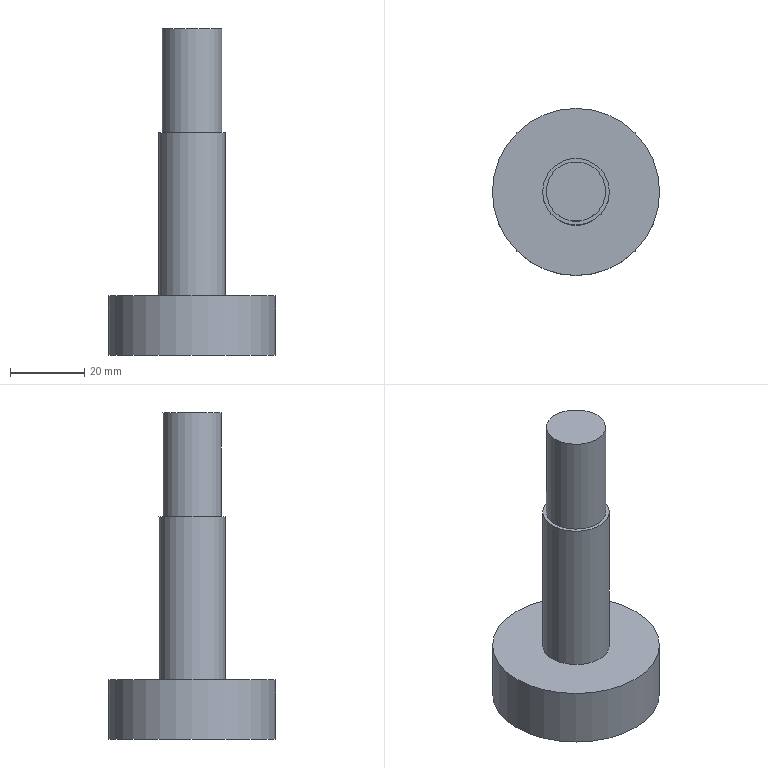Component | NX | VALVE_CORE | 1 solid | 7 faces | box 45 x 45 x 88 mm | volume 42273 mm3 | plane 4 | cylinder 3 | commonest cylinder face diameters 45 x1 18 x1 16 x1
STEP:
#1=CARTESIAN_POINT('',(0.,0.,0.));
#2=DIRECTION('',(0.,0.,1.));
#3=DIRECTION('',(1.,0.,0.));
#4=AXIS2_PLACEMENT_3D('',#1,#2,#3);
#5=CARTESIAN_POINT('',(90.249,-116.649,-76.615));
#6=VERTEX_POINT('',#5);
#7=CARTESIAN_POINT('',(81.249,-116.649,-76.615));
#8=DIRECTION('',(0.,0.,1.));
#9=DIRECTION('',(1.,0.,0.));
#10=AXIS2_PLACEMENT_3D('',#7,#8,#9);
#11=CIRCLE('',#10,9.);
#12=CARTESIAN_POINT('',(81.249,-116.649,-76.615));
#13=DIRECTION('',(0.,0.,1.));
#14=DIRECTION('',(1.,0.,0.));
#15=AXIS2_PLACEMENT_3D('',#12,#13,#14);
#16=PLANE('',#15);
#17=CARTESIAN_POINT('',(0.,0.));
#18=DIRECTION('',(1.,0.));
#19=AXIS2_PLACEMENT_2D('',#17,#18);
#20=CIRCLE('',#19,9.);
#21=(GEOMETRIC_REPRESENTATION_CONTEXT(2)PARAMETRIC_REPRESENTATION_CONTEXT()REPRESENTATION_CONTEXT('',''));
#22=DEFINITIONAL_REPRESENTATION('',(#20),#21);
#23=PCURVE('',#16,#22);
#24=CARTESIAN_POINT('',(81.249,-116.649,-76.615));
#25=DIRECTION('',(0.,0.,1.));
#26=DIRECTION('',(1.,0.,0.));
#27=AXIS2_PLACEMENT_3D('',#24,#25,#26);
#28=CYLINDRICAL_SURFACE('',#27,9.);
#29=CARTESIAN_POINT('',(0.,0.));
#30=DIRECTION('',(1.,0.));
#31=VECTOR('',#30,1.);
#32=LINE('',#29,#31);
#33=(GEOMETRIC_REPRESENTATION_CONTEXT(2)PARAMETRIC_REPRESENTATION_CONTEXT()REPRESENTATION_CONTEXT('',''));
#34=DEFINITIONAL_REPRESENTATION('',(#32),#33);
#35=PCURVE('',#28,#34);
#36=SURFACE_CURVE('',#11,(#23,#35),.PCURVE_S1.);
#37=EDGE_CURVE('',#6,#6,#36,.T.);
#38=ORIENTED_EDGE('',*,*,#37,.F.);
#39=EDGE_LOOP('',(#38));
#40=FACE_BOUND('',#39,.T.);
#41=CARTESIAN_POINT('',(103.749,-116.649,-76.615));
#42=VERTEX_POINT('',#41);
#43=CARTESIAN_POINT('',(81.249,-116.649,-76.615));
#44=DIRECTION('',(0.,0.,-1.));
#45=DIRECTION('',(1.,0.,0.));
#46=AXIS2_PLACEMENT_3D('',#43,#44,#45);
#47=CIRCLE('',#46,22.5);
#48=CARTESIAN_POINT('',(22.5,0.));
#49=CARTESIAN_POINT('',(22.5,-38.971));
#50=CARTESIAN_POINT('',(-11.25,-19.486));
#51=CARTESIAN_POINT('',(-45.,-0.));
#52=CARTESIAN_POINT('',(-11.25,19.486));
#53=CARTESIAN_POINT('',(22.5,38.971));
#54=CARTESIAN_POINT('',(22.5,0.));
#55=(BOUNDED_CURVE()B_SPLINE_CURVE(2,(#48,#49,#50,#51,#52,#53,#54),.UNSPECIFIED.,.T.,.F.)B_SPLINE_CURVE_WITH_KNOTS((1,2,2,2,2,1),(-2.094,0.,2.094,4.189,6.283,8.378),.UNSPECIFIED.)CURVE()GEOMETRIC_REPRESENTATION_ITEM()RATIONAL_B_SPLINE_CURVE((1.,0.5,1.,0.5,1.,0.5,1.))REPRESENTATION_ITEM(''));
#56=(GEOMETRIC_REPRESENTATION_CONTEXT(2)PARAMETRIC_REPRESENTATION_CONTEXT()REPRESENTATION_CONTEXT('',''));
#57=DEFINITIONAL_REPRESENTATION('',(#55),#56);
#58=PCURVE('',#16,#57);
#59=CARTESIAN_POINT('',(81.249,-116.649,-92.615));
#60=DIRECTION('',(0.,0.,1.));
#61=DIRECTION('',(1.,0.,0.));
#62=AXIS2_PLACEMENT_3D('',#59,#60,#61);
#63=CYLINDRICAL_SURFACE('',#62,22.5);
#64=CARTESIAN_POINT('',(6.283,16.));
#65=DIRECTION('',(-1.,0.));
#66=VECTOR('',#65,1.);
#67=LINE('',#64,#66);
#68=(GEOMETRIC_REPRESENTATION_CONTEXT(2)PARAMETRIC_REPRESENTATION_CONTEXT()REPRESENTATION_CONTEXT('',''));
#69=DEFINITIONAL_REPRESENTATION('',(#67),#68);
#70=PCURVE('',#63,#69);
#71=SURFACE_CURVE('',#47,(#58,#70),.PCURVE_S1.);
#72=EDGE_CURVE('',#42,#42,#71,.T.);
#73=ORIENTED_EDGE('',*,*,#72,.F.);
#74=EDGE_LOOP('',(#73));
#75=FACE_BOUND('',#74,.T.);
#76=ADVANCED_FACE('',(#40,#75),#16,.T.);
#77=CARTESIAN_POINT('',(103.749,-116.649,-92.615));
#78=VERTEX_POINT('',#77);
#79=CARTESIAN_POINT('',(81.249,-116.649,-92.615));
#80=DIRECTION('',(0.,0.,1.));
#81=DIRECTION('',(1.,0.,0.));
#82=AXIS2_PLACEMENT_3D('',#79,#80,#81);
#83=CIRCLE('',#82,22.5);
#84=CARTESIAN_POINT('',(81.249,-116.649,-92.615));
#85=DIRECTION('',(0.,0.,-1.));
#86=DIRECTION('',(-1.,0.,0.));
#87=AXIS2_PLACEMENT_3D('',#84,#85,#86);
#88=PLANE('',#87);
#89=CARTESIAN_POINT('',(-22.5,0.));
#90=CARTESIAN_POINT('',(-22.5,38.971));
#91=CARTESIAN_POINT('',(11.25,19.486));
#92=CARTESIAN_POINT('',(45.,0.));
#93=CARTESIAN_POINT('',(11.25,-19.486));
#94=CARTESIAN_POINT('',(-22.5,-38.971));
#95=CARTESIAN_POINT('',(-22.5,0.));
#96=(BOUNDED_CURVE()B_SPLINE_CURVE(2,(#89,#90,#91,#92,#93,#94,#95),.UNSPECIFIED.,.T.,.F.)B_SPLINE_CURVE_WITH_KNOTS((1,2,2,2,2,1),(-2.094,0.,2.094,4.189,6.283,8.378),.UNSPECIFIED.)CURVE()GEOMETRIC_REPRESENTATION_ITEM()RATIONAL_B_SPLINE_CURVE((1.,0.5,1.,0.5,1.,0.5,1.))REPRESENTATION_ITEM(''));
#97=(GEOMETRIC_REPRESENTATION_CONTEXT(2)PARAMETRIC_REPRESENTATION_CONTEXT()REPRESENTATION_CONTEXT('',''));
#98=DEFINITIONAL_REPRESENTATION('',(#96),#97);
#99=PCURVE('',#88,#98);
#100=CARTESIAN_POINT('',(0.,0.));
#101=DIRECTION('',(1.,0.));
#102=VECTOR('',#101,1.);
#103=LINE('',#100,#102);
#104=(GEOMETRIC_REPRESENTATION_CONTEXT(2)PARAMETRIC_REPRESENTATION_CONTEXT()REPRESENTATION_CONTEXT('',''));
#105=DEFINITIONAL_REPRESENTATION('',(#103),#104);
#106=PCURVE('',#63,#105);
#107=SURFACE_CURVE('',#83,(#99,#106),.PCURVE_S1.);
#108=EDGE_CURVE('',#78,#78,#107,.T.);
#109=ORIENTED_EDGE('',*,*,#108,.F.);
#110=EDGE_LOOP('',(#109));
#111=FACE_BOUND('',#110,.T.);
#112=ADVANCED_FACE('',(#111),#88,.T.);
#113=ORIENTED_EDGE('',*,*,#72,.T.);
#114=CARTESIAN_POINT('',(103.749,-116.649,-92.615));
#115=CARTESIAN_POINT('',(103.749,-116.649,-76.615));
#116=B_SPLINE_CURVE_WITH_KNOTS('',1,(#114,#115),.UNSPECIFIED.,.F.,.F.,(2,2),(0.,16.),.PIECEWISE_BEZIER_KNOTS.);
#117=CARTESIAN_POINT('',(0.,0.));
#118=DIRECTION('',(0.,1.));
#119=VECTOR('',#118,1.);
#120=LINE('',#117,#119);
#121=(GEOMETRIC_REPRESENTATION_CONTEXT(2)PARAMETRIC_REPRESENTATION_CONTEXT()REPRESENTATION_CONTEXT('',''));
#122=DEFINITIONAL_REPRESENTATION('',(#120),#121);
#123=PCURVE('',#63,#122);
#124=CARTESIAN_POINT('',(6.283,0.));
#125=DIRECTION('',(0.,1.));
#126=VECTOR('',#125,1.);
#127=LINE('',#124,#126);
#128=(GEOMETRIC_REPRESENTATION_CONTEXT(2)PARAMETRIC_REPRESENTATION_CONTEXT()REPRESENTATION_CONTEXT('',''));
#129=DEFINITIONAL_REPRESENTATION('',(#127),#128);
#130=PCURVE('',#63,#129);
#131=SEAM_CURVE('',#116,(#123,#130),.PCURVE_S1.);
#132=EDGE_CURVE('',#78,#42,#131,.T.);
#133=ORIENTED_EDGE('',*,*,#132,.F.);
#134=ORIENTED_EDGE('',*,*,#108,.T.);
#135=ORIENTED_EDGE('',*,*,#132,.T.);
#136=EDGE_LOOP('',(#113,#133,#134,#135));
#137=FACE_BOUND('',#136,.T.);
#138=ADVANCED_FACE('',(#137),#63,.T.);
#139=CARTESIAN_POINT('',(89.249,-116.649,-32.615));
#140=VERTEX_POINT('',#139);
#141=CARTESIAN_POINT('',(81.249,-116.649,-32.615));
#142=DIRECTION('',(0.,0.,1.));
#143=DIRECTION('',(1.,0.,0.));
#144=AXIS2_PLACEMENT_3D('',#141,#142,#143);
#145=CIRCLE('',#144,8.);
#146=CARTESIAN_POINT('',(81.249,-116.649,-32.615));
#147=DIRECTION('',(0.,0.,1.));
#148=DIRECTION('',(1.,0.,0.));
#149=AXIS2_PLACEMENT_3D('',#146,#147,#148);
#150=PLANE('',#149);
#151=CARTESIAN_POINT('',(0.,0.));
#152=DIRECTION('',(1.,0.));
#153=AXIS2_PLACEMENT_2D('',#151,#152);
#154=CIRCLE('',#153,8.);
#155=(GEOMETRIC_REPRESENTATION_CONTEXT(2)PARAMETRIC_REPRESENTATION_CONTEXT()REPRESENTATION_CONTEXT('',''));
#156=DEFINITIONAL_REPRESENTATION('',(#154),#155);
#157=PCURVE('',#150,#156);
#158=CARTESIAN_POINT('',(81.249,-116.649,-32.615));
#159=DIRECTION('',(0.,0.,1.));
#160=DIRECTION('',(1.,0.,0.));
#161=AXIS2_PLACEMENT_3D('',#158,#159,#160);
#162=CYLINDRICAL_SURFACE('',#161,8.);
#163=CARTESIAN_POINT('',(0.,0.));
#164=DIRECTION('',(1.,0.));
#165=VECTOR('',#164,1.);
#166=LINE('',#163,#165);
#167=(GEOMETRIC_REPRESENTATION_CONTEXT(2)PARAMETRIC_REPRESENTATION_CONTEXT()REPRESENTATION_CONTEXT('',''));
#168=DEFINITIONAL_REPRESENTATION('',(#166),#167);
#169=PCURVE('',#162,#168);
#170=SURFACE_CURVE('',#145,(#157,#169),.PCURVE_S1.);
#171=EDGE_CURVE('',#140,#140,#170,.T.);
#172=ORIENTED_EDGE('',*,*,#171,.F.);
#173=EDGE_LOOP('',(#172));
#174=FACE_BOUND('',#173,.T.);
#175=CARTESIAN_POINT('',(90.249,-116.649,-32.615));
#176=VERTEX_POINT('',#175);
#177=CARTESIAN_POINT('',(81.249,-116.649,-32.615));
#178=DIRECTION('',(0.,0.,1.));
#179=DIRECTION('',(1.,0.,0.));
#180=AXIS2_PLACEMENT_3D('',#177,#178,#179);
#181=CIRCLE('',#180,9.);
#182=CARTESIAN_POINT('',(0.,0.));
#183=DIRECTION('',(1.,0.));
#184=AXIS2_PLACEMENT_2D('',#182,#183);
#185=CIRCLE('',#184,9.);
#186=(GEOMETRIC_REPRESENTATION_CONTEXT(2)PARAMETRIC_REPRESENTATION_CONTEXT()REPRESENTATION_CONTEXT('',''));
#187=DEFINITIONAL_REPRESENTATION('',(#185),#186);
#188=PCURVE('',#150,#187);
#189=CARTESIAN_POINT('',(0.,44.));
#190=DIRECTION('',(1.,0.));
#191=VECTOR('',#190,1.);
#192=LINE('',#189,#191);
#193=(GEOMETRIC_REPRESENTATION_CONTEXT(2)PARAMETRIC_REPRESENTATION_CONTEXT()REPRESENTATION_CONTEXT('',''));
#194=DEFINITIONAL_REPRESENTATION('',(#192),#193);
#195=PCURVE('',#28,#194);
#196=SURFACE_CURVE('',#181,(#188,#195),.PCURVE_S1.);
#197=EDGE_CURVE('',#176,#176,#196,.T.);
#198=ORIENTED_EDGE('',*,*,#197,.T.);
#199=EDGE_LOOP('',(#198));
#200=FACE_BOUND('',#199,.T.);
#201=ADVANCED_FACE('',(#174,#200),#150,.T.);
#202=ORIENTED_EDGE('',*,*,#197,.F.);
#203=CARTESIAN_POINT('',(90.249,-116.649,-76.615));
#204=CARTESIAN_POINT('',(90.249,-116.649,-32.615));
#205=B_SPLINE_CURVE_WITH_KNOTS('',1,(#203,#204),.UNSPECIFIED.,.F.,.F.,(2,2),(0.,44.),.PIECEWISE_BEZIER_KNOTS.);
#206=CARTESIAN_POINT('',(0.,0.));
#207=DIRECTION('',(0.,1.));
#208=VECTOR('',#207,1.);
#209=LINE('',#206,#208);
#210=(GEOMETRIC_REPRESENTATION_CONTEXT(2)PARAMETRIC_REPRESENTATION_CONTEXT()REPRESENTATION_CONTEXT('',''));
#211=DEFINITIONAL_REPRESENTATION('',(#209),#210);
#212=PCURVE('',#28,#211);
#213=CARTESIAN_POINT('',(6.283,0.));
#214=DIRECTION('',(0.,1.));
#215=VECTOR('',#214,1.);
#216=LINE('',#213,#215);
#217=(GEOMETRIC_REPRESENTATION_CONTEXT(2)PARAMETRIC_REPRESENTATION_CONTEXT()REPRESENTATION_CONTEXT('',''));
#218=DEFINITIONAL_REPRESENTATION('',(#216),#217);
#219=PCURVE('',#28,#218);
#220=SEAM_CURVE('',#205,(#212,#219),.PCURVE_S1.);
#221=EDGE_CURVE('',#6,#176,#220,.T.);
#222=ORIENTED_EDGE('',*,*,#221,.F.);
#223=ORIENTED_EDGE('',*,*,#37,.T.);
#224=ORIENTED_EDGE('',*,*,#221,.T.);
#225=EDGE_LOOP('',(#202,#222,#223,#224));
#226=FACE_BOUND('',#225,.T.);
#227=ADVANCED_FACE('',(#226),#28,.T.);
#228=CARTESIAN_POINT('',(89.249,-116.649,-4.615));
#229=VERTEX_POINT('',#228);
#230=CARTESIAN_POINT('',(81.249,-116.649,-4.615));
#231=DIRECTION('',(0.,0.,1.));
#232=DIRECTION('',(1.,0.,0.));
#233=AXIS2_PLACEMENT_3D('',#230,#231,#232);
#234=CIRCLE('',#233,8.);
#235=CARTESIAN_POINT('',(81.249,-116.649,-4.615));
#236=DIRECTION('',(0.,0.,1.));
#237=DIRECTION('',(1.,0.,0.));
#238=AXIS2_PLACEMENT_3D('',#235,#236,#237);
#239=PLANE('',#238);
#240=CARTESIAN_POINT('',(0.,0.));
#241=DIRECTION('',(1.,0.));
#242=AXIS2_PLACEMENT_2D('',#240,#241);
#243=CIRCLE('',#242,8.);
#244=(GEOMETRIC_REPRESENTATION_CONTEXT(2)PARAMETRIC_REPRESENTATION_CONTEXT()REPRESENTATION_CONTEXT('',''));
#245=DEFINITIONAL_REPRESENTATION('',(#243),#244);
#246=PCURVE('',#239,#245);
#247=CARTESIAN_POINT('',(0.,28.));
#248=DIRECTION('',(1.,0.));
#249=VECTOR('',#248,1.);
#250=LINE('',#247,#249);
#251=(GEOMETRIC_REPRESENTATION_CONTEXT(2)PARAMETRIC_REPRESENTATION_CONTEXT()REPRESENTATION_CONTEXT('',''));
#252=DEFINITIONAL_REPRESENTATION('',(#250),#251);
#253=PCURVE('',#162,#252);
#254=SURFACE_CURVE('',#234,(#246,#253),.PCURVE_S1.);
#255=EDGE_CURVE('',#229,#229,#254,.T.);
#256=ORIENTED_EDGE('',*,*,#255,.T.);
#257=EDGE_LOOP('',(#256));
#258=FACE_BOUND('',#257,.T.);
#259=ADVANCED_FACE('',(#258),#239,.T.);
#260=ORIENTED_EDGE('',*,*,#255,.F.);
#261=CARTESIAN_POINT('',(89.249,-116.649,-32.615));
#262=CARTESIAN_POINT('',(89.249,-116.649,-4.615));
#263=B_SPLINE_CURVE_WITH_KNOTS('',1,(#261,#262),.UNSPECIFIED.,.F.,.F.,(2,2),(0.,28.),.PIECEWISE_BEZIER_KNOTS.);
#264=CARTESIAN_POINT('',(0.,0.));
#265=DIRECTION('',(0.,1.));
#266=VECTOR('',#265,1.);
#267=LINE('',#264,#266);
#268=(GEOMETRIC_REPRESENTATION_CONTEXT(2)PARAMETRIC_REPRESENTATION_CONTEXT()REPRESENTATION_CONTEXT('',''));
#269=DEFINITIONAL_REPRESENTATION('',(#267),#268);
#270=PCURVE('',#162,#269);
#271=CARTESIAN_POINT('',(6.283,0.));
#272=DIRECTION('',(0.,1.));
#273=VECTOR('',#272,1.);
#274=LINE('',#271,#273);
#275=(GEOMETRIC_REPRESENTATION_CONTEXT(2)PARAMETRIC_REPRESENTATION_CONTEXT()REPRESENTATION_CONTEXT('',''));
#276=DEFINITIONAL_REPRESENTATION('',(#274),#275);
#277=PCURVE('',#162,#276);
#278=SEAM_CURVE('',#263,(#270,#277),.PCURVE_S1.);
#279=EDGE_CURVE('',#140,#229,#278,.T.);
#280=ORIENTED_EDGE('',*,*,#279,.F.);
#281=ORIENTED_EDGE('',*,*,#171,.T.);
#282=ORIENTED_EDGE('',*,*,#279,.T.);
#283=EDGE_LOOP('',(#260,#280,#281,#282));
#284=FACE_BOUND('',#283,.T.);
#285=ADVANCED_FACE('',(#284),#162,.T.);
#286=CLOSED_SHELL('',(#76,#112,#138,#201,#227,#259,#285));
#287=MANIFOLD_SOLID_BREP('',#286);
#288=(LENGTH_UNIT()NAMED_UNIT(*)SI_UNIT(.MILLI.,.METRE.));
#289=UNCERTAINTY_MEASURE_WITH_UNIT(LENGTH_MEASURE(0.00001),#288,'','');
#290=(NAMED_UNIT(*)PLANE_ANGLE_UNIT()SI_UNIT($,.RADIAN.));
#291=(NAMED_UNIT(*)SI_UNIT($,.STERADIAN.)SOLID_ANGLE_UNIT());
#292=(GEOMETRIC_REPRESENTATION_CONTEXT(3)GLOBAL_UNCERTAINTY_ASSIGNED_CONTEXT((#289))GLOBAL_UNIT_ASSIGNED_CONTEXT((#288,#290,#291))REPRESENTATION_CONTEXT('',''));
#293=ADVANCED_BREP_SHAPE_REPRESENTATION('',(#4,#287),#292);